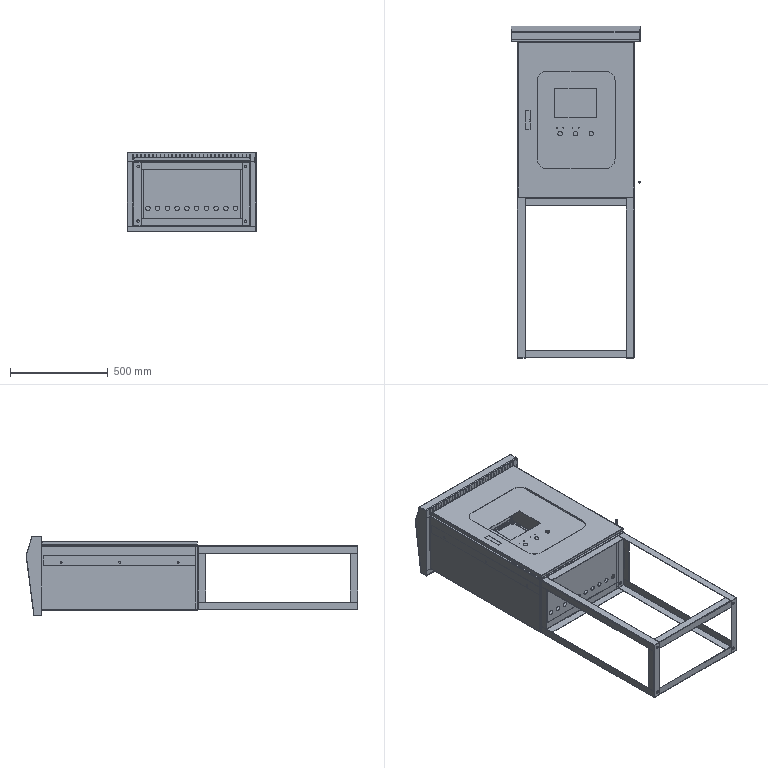Assembly | SolidWorks | mm | 42 component files | 42 solids | 1692 faces | box 662.32 x 1701.47 x 410 mm | volume 6257077 mm3 | plane 1073 | cylinder 561 | spline 34 | cone 12 | torus 12 | commonest cylinder face diameters 8 x164 3.2 x148 0.2 x67 23 x26 12.639 x16 4.2 x13 9 x12 6 x12
Bill of materials:
AEBox-BoxHinge | 3 |  | Flat rectangular leaf with a rolled cylindrical knuckle along one long edge. The knuckle is split into two end segments with a gap cut out in the middle. The leaf has two countersunk through-holes. Overall it looks like a single hinge leaf.
AEBox-DoorHinge | 3 |  | Sheet folded back on itself into a U/C (hairpin) cross-section with a large rounded bend. The two free edges are castellated, with rectangular tabs and notches that line up opposite each other across the opening.
BaseBracketDepth | 4 | 2.0mm Cold Rolled Plate | Narrow flat strip bent 90 degrees into an L-shaped bracket with a rounded bend. One leg has two round holes near its ends.
BaseBracketHeight | 4 | 2.0mm Cold Rolled Plate | Long straight angle profile with thin walls, roughly equal legs and a small rounded inside bend. No holes or cutouts are visible.
BaseBracketWidth | 4 | 2.0mm Cold Rolled Plate | Long straight thin-walled angle profile with an L-shaped cross-section and a rounded inside bend. No holes are visible. It looks very similar to unnamed part but is shown in a different orientation.
BottomPlate | 1 |  | Flat rectangular sheet panel. Along one long edge is a short offset return flange with an angled lip, giving a joggled or Z-like edge. The panel has a row of ten equal round holes and four smaller holes near the corners.
BottomPlateReinforcementBeam | 2 |  | Narrow rectangular sheet strip with a round hole near each end and a short 90-degree flange along one long edge, giving an L-shaped cross-section.
Box | 1 |  | Open U-shaped sheet channel or tray: a flat rectangular base with two tall parallel side walls. The top edges of the walls end in small inward return lips with angled tips. There are small holes or marks near the wall tops and on the base.
Column | 2 |  | Long formed sheet profile with a stepped hat/Z-like cross-section: a tall vertical leg, a horizontal top web, a downward leg, and an outward horizontal flange, with small rounded bends. One face has three small round holes spaced along its length.
Hinge1 | 3 |  | Plain hollow cylindrical tube or sleeve with a concentric round bore, about two and a half times as long as its outer diameter. The ends are flat.
Hinge2 | 3 |  | Solid stepped cylindrical pin: a larger-diameter section joined coaxially to a longer, smaller-diameter shank, with a flat shoulder between them. Both ends are flat.
InnerDoor | 1 |  | Thin flat rectangular plate. It has one large rectangular cutout, a row of three round holes below it, one small rounded-square hole near one side edge, and four tiny holes in pairs above the round holes.
M8X25WeldScrew | 3 |  | Headed cylindrical stud: a thin, flat, circular head on top of a straight shank with an external thread-like helical/ringed profile running its full length.
MountingPlate | 1 |  | Thin, flat rectangular plate with one small through-hole near each of its four corners.
OuterDoor | 1 |  | Thin, flat rectangular plate with a large central rounded-rectangle cutout and a small rectangular slot between the cutout and one long edge.
RainproofTopCover | 1 |  | Long formed sheet profile: a web with a kink, plus a top and a bottom flange that point the same way, giving an angled, channel-like cross-section.
TopCoverFrontSideBeam | 1 |  | Long thin-wall stepped Z-like profile rail with a row of evenly spaced, narrow vertical slots along the main web.
TopCoverLeftSealingPlate | 1 |  | Short formed sheet bracket. Its cross-section is a tall leg, a base and a small stepped return flange. One side outline is tapered or angled.
TopCoverRearSideBeam | 1 |  | Long thin-wall stepped Z-like rail: an upper leg, an offset step, a long web and a bottom flange, with no holes.
TopCoverRightSealingPlate | 1 |  | Short formed sheet bracket, apparently the mirror image of unnamed part: a tall leg, a base and a small stepped return flange, with a tapered side outline.
UpperBeam | 1 |  | Long thin-wall formed profile: a roughly 45-degree angled lip, a short vertical leg, a wide horizontal web and a long vertical leg turned the opposite way. The ends of the angled lip appear chamfered.
Mates:
1. coincident | Box-1 face at (-344.359, -450.131, 956.637) dir (0, -1, 0) | BottomPlate-1 face at (-44.359, -450.131, 792.387) dir (0, -1, 0)
2. coincident | UpperBeam-1 face at (-322.359, 327.869, 955.137) dir (-1, 0, 0) | Box-1 face at (-322.359, -45.131, 628.137) dir (1, 0, 0)
3. concentric | Box-1 face at (-309.359, 319.869, 638.137) dir (0, 0, -1) r 1 | MountingPlate-1 face at (-309.359, 319.869, 633.137) dir (0, 0, 1) r 4
4. concentric | Box-1 face at (220.641, 319.869, 638.137) dir (0, 0, -1) r 1 | MountingPlate-1 face at (220.641, 319.869, 633.137) dir (0, 0, 1) r 4
5. distance | Box-1 face at (-344.359, -45.131, 628.137) dir (-1, 0, 0) | RainproofTopCover-1 face at (-374.359, 400.274, 1005.066) dir (-1, 0, 0)
6. distance | RainproofTopCover-1 face at (-374.359, 351.369, 596.637) dir (0, 0, -1) | Box-1 face at (-44.359, -45.131, 626.637) dir (0, 0, -1)
7. coincident | RainproofTopCover-1 face at (-374.359, 400.274, 1005.066) dir (-1, 0, 0) | TopCoverLeftSealingPlate-1 face at (-374.359, 430.369, 908.696) dir (-1, 0, 0)
8. coincident | RainproofTopCover-1 face at (285.641, 400.178, 1005.037) dir (1, 0, 0) | TopCoverRightSealingPlate-1 face at (285.641, 430.369, 908.696) dir (1, 0, 0)
9. coincident | RainproofTopCover-1 face at (-374.359, 401.369, 1005.137) dir (0, 0, -1) | TopCoverLeftSealingPlate-1 face at (-372.859, 351.369, 1005.137) dir (0, 0, 1)
10. coincident | RainproofTopCover-1 face at (-374.359, 401.369, 1005.137) dir (0, 0, -1) | TopCoverRightSealingPlate-1 face at (285.641, 351.369, 1005.137) dir (0, 0, 1)
11. coincident | Box-1 face at (-342.859, -45.131, 628.137) dir (1, 0, 0) | Column-1 face at (-342.859, -48.631, 906.637) dir (-1, 0, 0)
12. coincident | Column-1 face at (-342.859, -438.631, 856.637) dir (0, -1, 0) | Column-2 face at (254.141, -438.631, 905.137) dir (0, -1, 0)
13. coincident | Column-1 face at (-330.359, -48.631, 906.637) dir (0, 0, 1) | Column-2 face at (241.641, -48.631, 906.637) dir (0, 0, 1)
14. coincident | Box-1 face at (254.141, -45.131, 628.137) dir (-1, 0, 0) | Column-2 face at (254.141, -48.631, 906.637) dir (1, 0, 0)
15. distance | Column-1 face at (-330.359, -48.631, 906.637) dir (0, 0, 1) | Box-1 face at (-44.359, -45.131, 956.637) dir (0, 0, 1)
16. concentric | Hinge1-1 face at (223.391, -322.131, 912.387) dir (0, -1, 0) r 5.75 | Hinge2-1 face at (223.391, -342.131, 912.387) dir (0, 1, 0) r 3
17. coincident | Hinge1-1 face at (223.391, -322.131, 912.387) dir (0, 1, 0) | Hinge2-1 face at (223.391, -322.131, 912.387) dir (0, -1, 0)
18. tangent | Column-2 face at (241.641, -48.631, 906.637) dir (0, 0, 1) | Hinge2-1 face at (223.391, -294.131, 912.387) dir (0, -1, 0) r 5.75
19. tangent | Column-2 face at (229.141, -48.631, 906.637) dir (-1, 0, 0) | Hinge2-1 face at (223.391, -294.131, 912.387) dir (0, -1, 0) r 5.75
20. distance | Hinge1-1 face at (223.391, -350.131, 912.387) dir (0, -1, 0) | BottomPlate-1 face at (-44.359, -450.131, 792.387) dir (0, -1, 0)
21. coincident | Hinge1-1 face at (229.391, -336.131, 906.387) dir (0, 0, -1) | InnerDoor-1 face at (-44.924, -53.131, 906.387) dir (0, 0, 1)
22. distance | InnerDoor-1 face at (-44.924, -418.131, 906.387) dir (0, -1, 0) | BottomPlate-1 face at (-44.359, -428.131, 792.387) dir (0, 1, 0)
23. distance | Hinge1-1 face at (224.076, -348.917, 500906.387) dir (1, 0, 0) | InnerDoor-1 face at (225.076, -53.131, 906.387) dir (1, 0, 0)
24. angle | Column-2 face at (241.641, -48.631, 888.137) dir (0, 0, 1) | InnerDoor-1 face at (-44.924, -53.131, 906.387) dir (0, 0, 1)
25. coincident | Box-1 face at (-44.359, -45.131, 956.637) dir (0, 0, 1) | AEBox-BoxHinge-1 face at (253.841, 219.869, 956.637) dir (0, 0, -1)
26. concentric | Box-1 edge at (247.641, 258.619, 956.637) dir (0, 0, 1) r 3.5 | AEBox-BoxHinge-1 edge at (247.641, 258.619, 956.637) dir (0, 0, -1) r 2.5
27. concentric | Box-1 face at (247.641, 241.119, 946.637) dir (0, 0, 1) r 3.5 | AEBox-BoxHinge-1 face at (247.641, 241.119, 958.137) dir (0, 0, -1) r 785.398
28. concentric | AEBox-DoorHinge-1 face at (247.811, 237.369, 968.597) dir (0, 1, 0) r 4.25 | AEBox-BoxHinge-1 face at (247.811, 263.119, 968.597) dir (0, -1, 0) r 4.25
29. distance | AEBox-DoorHinge-1 face at (247.811, 237.369, 965.847) dir (0, -1, 0) | AEBox-BoxHinge-1 face at (247.811, 236.619, 968.597) dir (0, 1, 0)
30. coincident | AEBox-DoorHinge-1 face at (252.561, 262.369, 974.347) dir (1, 0, 0) | OuterDoor-1 face at (252.561, -50.081, 980.547) dir (-1, 0, 0)
31. angle | BottomPlate-1 face at (-44.359, -448.631, 956.637) dir (0, 0, 1) | OuterDoor-1 face at (-42.939, -50.081, 980.547) dir (0, 0, 1)
32. coincident | BottomPlate-1 face at (-44.359, -448.631, 792.387) dir (0, 1, 0) | BottomPlateReinforcementBeam-1 face at (-317.359, -448.631, 792.387) dir (0, -1, 0)
33. concentric | BottomPlate-1 edge at (230.641, -448.631, 932.387) dir (0, 1, 0) r 6 | BottomPlateReinforcementBeam-2 edge at (230.641, -446.631, 932.387) dir (0, 1, 0) r 6.5
34. concentric | BottomPlate-1 edge at (-319.359, -448.631, 652.387) dir (0, 1, 0) r 6 | BottomPlateReinforcementBeam-1 edge at (-319.359, -446.631, 652.387) dir (0, 1, 0) r 6.5
35. coincident | Box-1 face at (-44.359, 359.869, 628.137) dir (0, 1, 0) | TopCoverLeftSealingPlate-1 face at (-374.359, 359.869, 908.696) dir (0, -1, 0)
36. coincident | TopCoverLeftSealingPlate-1 face at (-374.359, 351.369, 908.696) dir (0, -1, 0) | TopCoverRearSideBeam-1 face at (-44.359, 351.369, 612.387) dir (0, -1, 0)
37. coincident | RainproofTopCover-1 face at (-374.359, 351.369, 598.137) dir (0, 0, 1) | TopCoverRearSideBeam-1 face at (-44.359, 352.869, 598.137) dir (0, 0, -1)
38. coincident | TopCoverRightSealingPlate-1 face at (284.141, 430.369, 908.696) dir (-1, 0, 0) | TopCoverRearSideBeam-1 face at (284.141, 351.369, 626.637) dir (1, 0, 0)
39. coincident | RainproofTopCover-1 face at (-374.359, 401.369, 1005.137) dir (0, 0, -1) | TopCoverFrontSideBeam-1 face at (-44.359, 352.869, 1005.137) dir (0, 0, 1)
40. coincident | TopCoverLeftSealingPlate-1 face at (-374.359, 351.369, 908.696) dir (0, -1, 0) | TopCoverFrontSideBeam-1 face at (-44.359, 351.369, 980.887) dir (0, -1, 0)
41. coincident | TopCoverRightSealingPlate-1 face at (284.141, 430.369, 908.696) dir (-1, 0, 0) | TopCoverFrontSideBeam-1 face at (284.141, 351.369, 1005.137) dir (1, 0, 0)
42. concentric | AEBox-DoorHinge-1 face at (252.561, 257.419, 965.547) dir (-1, 0, 0) r 1.2 | OuterDoor-1 face at (244.561, 257.419, 965.547) dir (1, 0, 0) r 1.6
43. coincident | Box-1 face at (254.141, -45.131, 628.137) dir (-1, 0, 0) | BottomPlate-1 face at (254.141, -450.131, 956.637) dir (1, 0, 0)
44. coincident | TopCoverLeftSealingPlate-1 face at (-374.359, 361.369, 908.696) dir (0, 1, 0) | TopCoverRightSealingPlate-1 face at (284.141, 361.369, 908.696) dir (0, 1, 0)
45. coincident | Column-1 face at (-342.859, -438.631, 905.137) dir (0, -1, 0) | BottomPlateReinforcementBeam-1 face at (-342.359, -438.631, 637.387) dir (0, 1, 0)
46. coincident | Box-1 face at (-44.359, -45.131, 956.637) dir (0, 0, 1) | UpperBeam-1 face at (-44.359, 343.869, 956.637) dir (0, 0, 1)
47. coincident | Box-1 face at (-44.359, 358.369, 628.137) dir (0, -1, 0) | UpperBeam-1 face at (-44.359, 358.369, 956.637) dir (0, -1, 0)
48. coincident | Box-1 face at (-44.359, -45.131, 628.137) dir (0, 0, 1) | BottomPlate-1 face at (-342.859, -450.131, 628.137) dir (0, 0, -1)
49. concentric | BottomPlate-1 face at (230.641, -458.631, 932.387) dir (0, 1, 0) r 6 | BaseBracketAssembly-1/BaseBracketDepth-10 edge at (230.641, -452.131, 932.387) dir (0, -1, 0) r 6.32
50. coincident | BottomPlate-1 face at (-44.359, -450.131, 792.387) dir (0, -1, 0) | BaseBracketAssembly-1/BaseBracketDepth-10 face at (255.641, -450.131, 917.387) dir (0, 1, 0)
51. parallel | Box-1 face at (255.641, -45.131, 628.137) dir (1, 0, 0) | BaseBracketAssembly-1/BaseBracketDepth-10 face at (255.641, -490.131, 917.387) dir (1, 0, 0)
52. parallel | AEBox-BoxHinge-1 edge at (242.508, 263.119, 969.304) dir (0, -1, 0) | OuterDoor-1 edge at (252.561, 347.419, 963.547) dir (0, -1, 0)
53. coincident | Box-1 face at (254.141, -45.131, 628.137) dir (-1, 0, 0) | M8X25WeldScrew-2 face at (254.141, -373.871, 815.471) dir (1, 0, 0)
54. coincident | InnerDoor-1 face at (-44.924, -53.131, 904.887) dir (0, 0, -1) | M8X25WeldScrew-1 face at (182.274, -348.056, 904.887) dir (0, 0, 1)
55. coincident | OuterDoor-1 face at (-42.939, -50.081, 978.547) dir (0, 0, -1) | M8X25WeldScrew-3 face at (283.115, -368.839, 978.547) dir (0, 0, 1)
56. coincident | BaseBracketHeight-1 face at (-20, 20, 410) dir (-1, 0, 0) | BaseBracketWidth-1 face at (-20, 20, -370) dir (-1, 0, 0)
57. coincident | BaseBracketHeight-1 face at (-17.5, -17.5, -410) dir (0, 0, -1) | BaseBracketWidth-1 face at (-20, 20, -410) dir (0, 0, -1)
58. coincident | BaseBracketHeight-1 face at (-20, -20, 410) dir (0, -1, 0) | BaseBracketDepth-6 face at (20, -20, 370) dir (0, -1, 0)
59. coincident | BaseBracketHeight-1 face at (20, -18, 410) dir (1, 0, 0) | BaseBracketDepth-6 face at (20, -17.5, 408) dir (-1, 0, 0)
60. coincident | BaseBracketHeight-1 face at (-17.5, -17.5, 410) dir (0, 0, 1) | BaseBracketDepth-6 face at (20, -20, 410) dir (0, 0, 1)
61. coincident | BaseBracketWidth-1 face at (-20, 20, -410) dir (0, 0, -1) | BaseBracketDepth-7 face at (270, -20, -410) dir (0, 0, -1)
62. coincident | BaseBracketHeight-1 face at (20, -18, 410) dir (1, 0, 0) | BaseBracketDepth-7 face at (20, -17.5, -407.5) dir (-1, 0, 0)
63. coincident | BaseBracketHeight-1 face at (-20, 20, 410) dir (0, 1, 0) | BaseBracketWidth-1 face at (-17.5, 20, -408) dir (0, -1, 0)
64. coincident | BaseBracketDepth-6 face at (20, -20, 410) dir (0, 0, 1) | BaseBracketWidth-6 face at (270, 540, 410) dir (0, 0, 1)
65. coincident | BaseBracketDepth-6 face at (20, 20, 408) dir (0, 1, 0) | BaseBracketWidth-5 face at (-18, 20, 407.5) dir (0, -1, 0)
66. coincident | BaseBracketDepth-6 face at (20, -20, 410) dir (0, 0, 1) | BaseBracketWidth-5 face at (-20, 540, 410) dir (0, 0, 1)
67. coincident | BaseBracketHeight-1 face at (-20, 20, 410) dir (-1, 0, 0) | BaseBracketWidth-5 face at (-20, 540, 370) dir (-1, 0, 0)
68. coincident | BaseBracketWidth-1 face at (-20, 20, -370) dir (-1, 0, 0) | BaseBracketHeight-2 face at (-20, 580, 410) dir (-1, 0, 0)
69. coincident | BaseBracketWidth-1 face at (-17.5, 540, -407.5) dir (0, 1, 0) | BaseBracketHeight-2 face at (-18, 540, 410) dir (0, -1, 0)
70. coincident | BaseBracketWidth-1 face at (-20, 20, -410) dir (0, 0, -1) | BaseBracketHeight-2 face at (-17.5, 577.5, -410) dir (0, 0, -1)
71. coincident | BaseBracketHeight-3 face at (310, 580, 410) dir (0, 1, 0) | BaseBracketDepth-9 face at (20, 580, -370) dir (0, 1, 0)
72. coincident | BaseBracketHeight-3 face at (270, 578, 410) dir (-1, 0, 0) | BaseBracketDepth-9 face at (270, 577.5, -407.5) dir (1, 0, 0)
73. coincident | BaseBracketWidth-6 face at (270, 540, 410) dir (0, 0, 1) | BaseBracketDepth-10 face at (270, 580, 410) dir (0, 0, 1)
74. coincident | BaseBracketHeight-3 face at (310, 580, 410) dir (0, 1, 0) | BaseBracketDepth-10 face at (270, 580, 370) dir (0, 1, 0)
75. coincident | BaseBracketHeight-3 face at (270, 578, 410) dir (-1, 0, 0) | BaseBracketDepth-10 face at (270, 577.5, 408) dir (1, 0, 0)
76. coincident | BaseBracketDepth-7 face at (270, -20, -370) dir (0, -1, 0) | BaseBracketHeight-4 face at (270, -20, 410) dir (0, -1, 0)
77. coincident | BaseBracketDepth-7 face at (270, -20, -410) dir (0, 0, -1) | BaseBracketHeight-4 face at (307.5, -18, -410) dir (0, 0, -1)
78. coincident | BaseBracketHeight-3 face at (310, 540, 410) dir (1, 0, 0) | BaseBracketHeight-4 face at (310, -20, 410) dir (1, 0, 0)
79. coincident | BaseBracketDepth-7 face at (270, -20, -410) dir (0, 0, -1) | BaseBracketWidth-7 face at (270, 20, -410) dir (0, 0, -1)
80. coincident | BaseBracketHeight-4 face at (310, -20, 410) dir (1, 0, 0) | BaseBracketWidth-7 face at (310, 20, -410) dir (1, 0, 0)
81. coincident | BaseBracketDepth-7 face at (270, 20, -408) dir (0, 1, 0) | BaseBracketWidth-7 face at (308, 20, -407.5) dir (0, -1, 0)
82. coincident | BaseBracketWidth-6 face at (310, 540, 410) dir (1, 0, 0) | BaseBracketHeight-4 face at (310, -20, 410) dir (1, 0, 0)
83. coincident | BaseBracketDepth-6 face at (20, -20, 410) dir (0, 0, 1) | BaseBracketWidth-6 face at (270, 540, 410) dir (0, 0, 1)
84. coincident | BaseBracketDepth-6 face at (20, 20, 408) dir (0, 1, 0) | BaseBracketWidth-6 face at (307.5, 20, 407.5) dir (0, -1, 0)
85. coincident | BaseBracketHeight-2 face at (20, 580, 410) dir (0, 1, 0) | BaseBracketDepth-9 face at (20, 580, -370) dir (0, 1, 0)
86. coincident | BaseBracketHeight-2 face at (-18, 580, 410) dir (1, 0, 0) | BaseBracketDepth-9 face at (-18, 540, -410) dir (-1, 0, 0)
87. coincident | BaseBracketHeight-1 face at (-20, -20, 410) dir (0, -1, 0) | BaseBracketDepth-7 face at (270, -20, -370) dir (0, -1, 0)
88. coincident | BaseBracketDepth-9 face at (20, 580, -410) dir (0, 0, -1) | BaseBracketWidth-7 face at (270, 20, -410) dir (0, 0, -1)